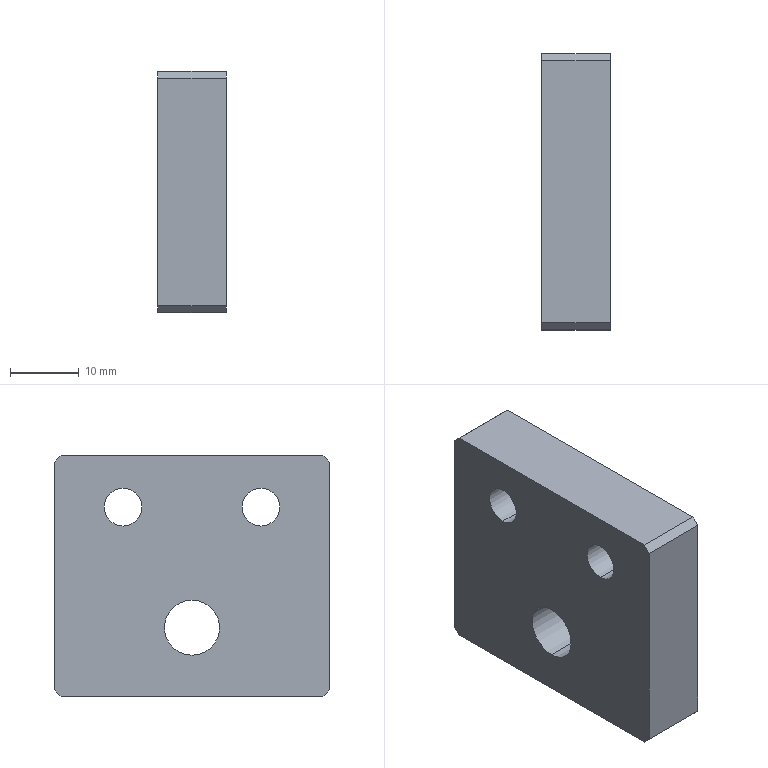Component | SolidWorks | XT-1-23-2-1 | 1 solid | 22 faces | box 10 x 40 x 35 mm | volume 12411 mm3 | plane 12 | cylinder 10 | commonest cylinder face diameters 10 x4 5.5 x4 8 x2
build123d program:
from build123d import *

# Parameters (mm, degrees)
SKETCH1_W                                       = 35
SKETCH1_H                                       = 40
BOSS_EXTRUDE1_DEPTH                             = 10
M5_HEX_SOCKET_HEAD_CAP_SCREW_CBORE1_D           = 5.5
M5_HEX_SOCKET_HEAD_CAP_SCREW_CBORE1_CBORE_D     = 10
M5_HEX_SOCKET_HEAD_CAP_SCREW_CBORE1_CBORE_DEPTH = 5.4
M8_TAPPED_HOLE1_D                               = 8
CHAMFER1_SIZE                                   = 1


with BuildPart() as part:
    # Sketch1 → Boss-Extrude1 (new body)
    with BuildSketch(Plane.XY):
        with Locations((17.5, -20)):
            Rectangle(SKETCH1_W, SKETCH1_H)
    extrude(amount=BOSS_EXTRUDE1_DEPTH)

    # M5 Hex Socket Head Cap Screw CBORE1 (through all)
    with Locations(Plane.XY.offset(10)):
        with Locations((7.5, -10), (7.5, -30)):
            CounterBoreHole(M5_HEX_SOCKET_HEAD_CAP_SCREW_CBORE1_D / 2, M5_HEX_SOCKET_HEAD_CAP_SCREW_CBORE1_CBORE_D / 2, M5_HEX_SOCKET_HEAD_CAP_SCREW_CBORE1_CBORE_DEPTH)

    # M8 Tapped Hole1 (through all)
    with Locations(Plane.XY.offset(10)):
        with Locations((25, -20)):
            Hole(M8_TAPPED_HOLE1_D / 2)

    # Chamfer1
    chamfer1_edges = [part.edges().sort_by_distance(p)[0] for p in [
        (0, 0, 5),
        (35, 0, 5),
        (35, -40, 5),
        (0, -40, 5),
    ]]
    chamfer(chamfer1_edges, length=CHAMFER1_SIZE)


solid = part.part

# Placed as in the assembly
solid = solid.moved(Location((587.283, -98.615, 20.5), (0, 90, 0)))
STEP:
#1=CARTESIAN_POINT('',(23.121,-4.67,-0.01969));
#2=VERTEX_POINT('',#1);
#3=CARTESIAN_POINT('',(23.121,-4.67,-0.3346));
#4=VERTEX_POINT('',#3);
#5=CARTESIAN_POINT('',(23.121,-4.67,-0.1772));
#6=DIRECTION('',(1.,-0.,0.));
#7=DIRECTION('',(0.,0.,-1.));
#8=AXIS2_PLACEMENT_3D('',#5,#6,#7);
#9=CIRCLE('',#8,0.1575);
#10=EDGE_CURVE('',#2,#4,#9,.T.);
#11=ORIENTED_EDGE('',*,*,#10,.F.);
#12=CARTESIAN_POINT('',(23.515,-4.67,-0.01969));
#13=VERTEX_POINT('',#12);
#14=CARTESIAN_POINT('',(23.515,-4.67,-0.01969));
#15=DIRECTION('',(1.,-0.,0.));
#16=VECTOR('',#15,39.37);
#17=LINE('',#14,#16);
#18=EDGE_CURVE('',#2,#13,#17,.T.);
#19=ORIENTED_EDGE('',*,*,#18,.T.);
#20=CARTESIAN_POINT('',(23.515,-4.67,-0.3346));
#21=VERTEX_POINT('',#20);
#22=CARTESIAN_POINT('',(23.515,-4.67,-0.1772));
#23=DIRECTION('',(1.,-0.,0.));
#24=DIRECTION('',(0.,0.,-1.));
#25=AXIS2_PLACEMENT_3D('',#22,#23,#24);
#26=CIRCLE('',#25,0.1575);
#27=EDGE_CURVE('',#13,#21,#26,.T.);
#28=ORIENTED_EDGE('',*,*,#27,.T.);
#29=CARTESIAN_POINT('',(23.515,-4.67,-0.3346));
#30=DIRECTION('',(1.,-0.,0.));
#31=VECTOR('',#30,39.37);
#32=LINE('',#29,#31);
#33=EDGE_CURVE('',#4,#21,#32,.T.);
#34=ORIENTED_EDGE('',*,*,#33,.F.);
#35=EDGE_LOOP('',(#11,#19,#28,#34));
#36=FACE_OUTER_BOUND('',#35,.T.);
#37=CARTESIAN_POINT('',(23.515,-4.67,-0.1772));
#38=DIRECTION('',(1.,-0.,0.));
#39=DIRECTION('',(0.,0.,-1.));
#40=AXIS2_PLACEMENT_3D('',#37,#38,#39);
#41=CYLINDRICAL_SURFACE('',#40,0.1575);
#42=ADVANCED_FACE('',(#36),#41,.F.);
#43=CARTESIAN_POINT('',(23.302,-4.276,0.7087));
#44=VERTEX_POINT('',#43);
#45=CARTESIAN_POINT('',(23.302,-4.276,0.315));
#46=VERTEX_POINT('',#45);
#47=CARTESIAN_POINT('',(23.302,-4.276,0.5118));
#48=DIRECTION('',(1.,-0.,0.));
#49=DIRECTION('',(0.,0.,-1.));
#50=AXIS2_PLACEMENT_3D('',#47,#48,#49);
#51=CIRCLE('',#50,0.1969);
#52=EDGE_CURVE('',#44,#46,#51,.T.);
#53=ORIENTED_EDGE('',*,*,#52,.F.);
#54=CARTESIAN_POINT('',(23.515,-4.276,0.7087));
#55=VERTEX_POINT('',#54);
#56=CARTESIAN_POINT('',(23.515,-4.276,0.7087));
#57=DIRECTION('',(1.,-0.,0.));
#58=VECTOR('',#57,39.37);
#59=LINE('',#56,#58);
#60=EDGE_CURVE('',#44,#55,#59,.T.);
#61=ORIENTED_EDGE('',*,*,#60,.T.);
#62=CARTESIAN_POINT('',(23.515,-4.276,0.315));
#63=VERTEX_POINT('',#62);
#64=CARTESIAN_POINT('',(23.515,-4.276,0.5118));
#65=DIRECTION('',(1.,-0.,0.));
#66=DIRECTION('',(0.,0.,-1.));
#67=AXIS2_PLACEMENT_3D('',#64,#65,#66);
#68=CIRCLE('',#67,0.1969);
#69=EDGE_CURVE('',#55,#63,#68,.T.);
#70=ORIENTED_EDGE('',*,*,#69,.T.);
#71=CARTESIAN_POINT('',(23.515,-4.276,0.315));
#72=DIRECTION('',(1.,-0.,0.));
#73=VECTOR('',#72,39.37);
#74=LINE('',#71,#73);
#75=EDGE_CURVE('',#46,#63,#74,.T.);
#76=ORIENTED_EDGE('',*,*,#75,.F.);
#77=EDGE_LOOP('',(#53,#61,#70,#76));
#78=FACE_OUTER_BOUND('',#77,.T.);
#79=CARTESIAN_POINT('',(23.515,-4.276,0.5118));
#80=DIRECTION('',(1.,-0.,0.));
#81=DIRECTION('',(0.,0.,-1.));
#82=AXIS2_PLACEMENT_3D('',#79,#80,#81);
#83=CYLINDRICAL_SURFACE('',#82,0.1969);
#84=ADVANCED_FACE('',(#78),#83,.F.);
#85=CARTESIAN_POINT('',(23.121,-4.276,0.6201));
#86=VERTEX_POINT('',#85);
#87=CARTESIAN_POINT('',(23.121,-4.276,0.4035));
#88=VERTEX_POINT('',#87);
#89=CARTESIAN_POINT('',(23.121,-4.276,0.5118));
#90=DIRECTION('',(1.,-0.,0.));
#91=DIRECTION('',(0.,0.,-1.));
#92=AXIS2_PLACEMENT_3D('',#89,#90,#91);
#93=CIRCLE('',#92,0.1083);
#94=EDGE_CURVE('',#86,#88,#93,.T.);
#95=ORIENTED_EDGE('',*,*,#94,.F.);
#96=CARTESIAN_POINT('',(23.302,-4.276,0.6201));
#97=VERTEX_POINT('',#96);
#98=CARTESIAN_POINT('',(23.515,-4.276,0.6201));
#99=DIRECTION('',(1.,-0.,0.));
#100=VECTOR('',#99,39.37);
#101=LINE('',#98,#100);
#102=EDGE_CURVE('',#86,#97,#101,.T.);
#103=ORIENTED_EDGE('',*,*,#102,.T.);
#104=CARTESIAN_POINT('',(23.302,-4.276,0.4035));
#105=VERTEX_POINT('',#104);
#106=CARTESIAN_POINT('',(23.302,-4.276,0.5118));
#107=DIRECTION('',(1.,-0.,0.));
#108=DIRECTION('',(0.,0.,-1.));
#109=AXIS2_PLACEMENT_3D('',#106,#107,#108);
#110=CIRCLE('',#109,0.1083);
#111=EDGE_CURVE('',#97,#105,#110,.T.);
#112=ORIENTED_EDGE('',*,*,#111,.T.);
#113=CARTESIAN_POINT('',(23.515,-4.276,0.4035));
#114=DIRECTION('',(1.,-0.,0.));
#115=VECTOR('',#114,39.37);
#116=LINE('',#113,#115);
#117=EDGE_CURVE('',#88,#105,#116,.T.);
#118=ORIENTED_EDGE('',*,*,#117,.F.);
#119=EDGE_LOOP('',(#95,#103,#112,#118));
#120=FACE_OUTER_BOUND('',#119,.T.);
#121=CARTESIAN_POINT('',(23.515,-4.276,0.5118));
#122=DIRECTION('',(1.,-0.,0.));
#123=DIRECTION('',(0.,0.,-1.));
#124=AXIS2_PLACEMENT_3D('',#121,#122,#123);
#125=CYLINDRICAL_SURFACE('',#124,0.1083);
#126=ADVANCED_FACE('',(#120),#125,.F.);
#127=CARTESIAN_POINT('',(23.302,-5.064,0.7087));
#128=VERTEX_POINT('',#127);
#129=CARTESIAN_POINT('',(23.302,-5.064,0.315));
#130=VERTEX_POINT('',#129);
#131=CARTESIAN_POINT('',(23.302,-5.064,0.5118));
#132=DIRECTION('',(1.,-0.,0.));
#133=DIRECTION('',(0.,0.,-1.));
#134=AXIS2_PLACEMENT_3D('',#131,#132,#133);
#135=CIRCLE('',#134,0.1969);
#136=EDGE_CURVE('',#128,#130,#135,.T.);
#137=ORIENTED_EDGE('',*,*,#136,.F.);
#138=CARTESIAN_POINT('',(23.515,-5.064,0.7087));
#139=VERTEX_POINT('',#138);
#140=CARTESIAN_POINT('',(23.515,-5.064,0.7087));
#141=DIRECTION('',(1.,-0.,0.));
#142=VECTOR('',#141,39.37);
#143=LINE('',#140,#142);
#144=EDGE_CURVE('',#128,#139,#143,.T.);
#145=ORIENTED_EDGE('',*,*,#144,.T.);
#146=CARTESIAN_POINT('',(23.515,-5.064,0.315));
#147=VERTEX_POINT('',#146);
#148=CARTESIAN_POINT('',(23.515,-5.064,0.5118));
#149=DIRECTION('',(1.,-0.,0.));
#150=DIRECTION('',(0.,0.,-1.));
#151=AXIS2_PLACEMENT_3D('',#148,#149,#150);
#152=CIRCLE('',#151,0.1969);
#153=EDGE_CURVE('',#139,#147,#152,.T.);
#154=ORIENTED_EDGE('',*,*,#153,.T.);
#155=CARTESIAN_POINT('',(23.515,-5.064,0.315));
#156=DIRECTION('',(1.,-0.,0.));
#157=VECTOR('',#156,39.37);
#158=LINE('',#155,#157);
#159=EDGE_CURVE('',#130,#147,#158,.T.);
#160=ORIENTED_EDGE('',*,*,#159,.F.);
#161=EDGE_LOOP('',(#137,#145,#154,#160));
#162=FACE_OUTER_BOUND('',#161,.T.);
#163=CARTESIAN_POINT('',(23.515,-5.064,0.5118));
#164=DIRECTION('',(1.,-0.,0.));
#165=DIRECTION('',(0.,0.,-1.));
#166=AXIS2_PLACEMENT_3D('',#163,#164,#165);
#167=CYLINDRICAL_SURFACE('',#166,0.1969);
#168=ADVANCED_FACE('',(#162),#167,.F.);
#169=CARTESIAN_POINT('',(23.121,-5.064,0.6201));
#170=VERTEX_POINT('',#169);
#171=CARTESIAN_POINT('',(23.121,-5.064,0.4035));
#172=VERTEX_POINT('',#171);
#173=CARTESIAN_POINT('',(23.121,-5.064,0.5118));
#174=DIRECTION('',(1.,-0.,0.));
#175=DIRECTION('',(0.,0.,-1.));
#176=AXIS2_PLACEMENT_3D('',#173,#174,#175);
#177=CIRCLE('',#176,0.1083);
#178=EDGE_CURVE('',#170,#172,#177,.T.);
#179=ORIENTED_EDGE('',*,*,#178,.F.);
#180=CARTESIAN_POINT('',(23.302,-5.064,0.6201));
#181=VERTEX_POINT('',#180);
#182=CARTESIAN_POINT('',(23.515,-5.064,0.6201));
#183=DIRECTION('',(1.,-0.,0.));
#184=VECTOR('',#183,39.37);
#185=LINE('',#182,#184);
#186=EDGE_CURVE('',#170,#181,#185,.T.);
#187=ORIENTED_EDGE('',*,*,#186,.T.);
#188=CARTESIAN_POINT('',(23.302,-5.064,0.4035));
#189=VERTEX_POINT('',#188);
#190=CARTESIAN_POINT('',(23.302,-5.064,0.5118));
#191=DIRECTION('',(1.,-0.,0.));
#192=DIRECTION('',(0.,0.,-1.));
#193=AXIS2_PLACEMENT_3D('',#190,#191,#192);
#194=CIRCLE('',#193,0.1083);
#195=EDGE_CURVE('',#181,#189,#194,.T.);
#196=ORIENTED_EDGE('',*,*,#195,.T.);
#197=CARTESIAN_POINT('',(23.515,-5.064,0.4035));
#198=DIRECTION('',(1.,-0.,0.));
#199=VECTOR('',#198,39.37);
#200=LINE('',#197,#199);
#201=EDGE_CURVE('',#172,#189,#200,.T.);
#202=ORIENTED_EDGE('',*,*,#201,.F.);
#203=EDGE_LOOP('',(#179,#187,#196,#202));
#204=FACE_OUTER_BOUND('',#203,.T.);
#205=CARTESIAN_POINT('',(23.515,-5.064,0.5118));
#206=DIRECTION('',(1.,-0.,0.));
#207=DIRECTION('',(0.,0.,-1.));
#208=AXIS2_PLACEMENT_3D('',#205,#206,#207);
#209=CYLINDRICAL_SURFACE('',#208,0.1083);
#210=ADVANCED_FACE('',(#204),#209,.F.);
#211=CARTESIAN_POINT('',(23.121,-3.922,0.8071));
#212=VERTEX_POINT('',#211);
#213=CARTESIAN_POINT('',(23.121,-5.418,0.8071));
#214=VERTEX_POINT('',#213);
#215=CARTESIAN_POINT('',(23.121,-3.882,0.8071));
#216=DIRECTION('',(-0.,-1.,-0.));
#217=VECTOR('',#216,39.37);
#218=LINE('',#215,#217);
#219=EDGE_CURVE('',#212,#214,#218,.T.);
#220=ORIENTED_EDGE('',*,*,#219,.T.);
#221=CARTESIAN_POINT('',(23.515,-5.418,0.8071));
#222=VERTEX_POINT('',#221);
#223=CARTESIAN_POINT('',(23.515,-5.418,0.8071));
#224=DIRECTION('',(1.,-0.,0.));
#225=VECTOR('',#224,39.37);
#226=LINE('',#223,#225);
#227=EDGE_CURVE('',#214,#222,#226,.T.);
#228=ORIENTED_EDGE('',*,*,#227,.T.);
#229=CARTESIAN_POINT('',(23.515,-3.922,0.8071));
#230=VERTEX_POINT('',#229);
#231=CARTESIAN_POINT('',(23.515,-3.882,0.8071));
#232=DIRECTION('',(-0.,-1.,-0.));
#233=VECTOR('',#232,39.37);
#234=LINE('',#231,#233);
#235=EDGE_CURVE('',#230,#222,#234,.T.);
#236=ORIENTED_EDGE('',*,*,#235,.F.);
#237=CARTESIAN_POINT('',(23.515,-3.922,0.8071));
#238=DIRECTION('',(-1.,0.,0.));
#239=VECTOR('',#238,39.37);
#240=LINE('',#237,#239);
#241=EDGE_CURVE('',#230,#212,#240,.T.);
#242=ORIENTED_EDGE('',*,*,#241,.T.);
#243=EDGE_LOOP('',(#220,#228,#236,#242));
#244=FACE_OUTER_BOUND('',#243,.T.);
#245=CARTESIAN_POINT('',(23.515,-3.882,0.8071));
#246=DIRECTION('',(0.,0.,-1.));
#247=DIRECTION('',(0.,1.,0.));
#248=AXIS2_PLACEMENT_3D('',#245,#246,#247);
#249=PLANE('',#248);
#250=ADVANCED_FACE('',(#244),#249,.F.);
#251=CARTESIAN_POINT('',(23.515,-5.457,0.7677));
#252=VERTEX_POINT('',#251);
#253=CARTESIAN_POINT('',(23.515,-5.457,-0.5315));
#254=VERTEX_POINT('',#253);
#255=CARTESIAN_POINT('',(23.515,-5.457,0.8071));
#256=DIRECTION('',(0.,0.,-1.));
#257=VECTOR('',#256,39.37);
#258=LINE('',#255,#257);
#259=EDGE_CURVE('',#252,#254,#258,.T.);
#260=ORIENTED_EDGE('',*,*,#259,.F.);
#261=CARTESIAN_POINT('',(23.121,-5.457,0.7677));
#262=VERTEX_POINT('',#261);
#263=CARTESIAN_POINT('',(23.515,-5.457,0.7677));
#264=DIRECTION('',(-1.,0.,0.));
#265=VECTOR('',#264,39.37);
#266=LINE('',#263,#265);
#267=EDGE_CURVE('',#252,#262,#266,.T.);
#268=ORIENTED_EDGE('',*,*,#267,.T.);
#269=CARTESIAN_POINT('',(23.121,-5.457,-0.5315));
#270=VERTEX_POINT('',#269);
#271=CARTESIAN_POINT('',(23.121,-5.457,0.8071));
#272=DIRECTION('',(0.,0.,-1.));
#273=VECTOR('',#272,39.37);
#274=LINE('',#271,#273);
#275=EDGE_CURVE('',#262,#270,#274,.T.);
#276=ORIENTED_EDGE('',*,*,#275,.T.);
#277=CARTESIAN_POINT('',(23.515,-5.457,-0.5315));
#278=DIRECTION('',(1.,-0.,0.));
#279=VECTOR('',#278,39.37);
#280=LINE('',#277,#279);
#281=EDGE_CURVE('',#270,#254,#280,.T.);
#282=ORIENTED_EDGE('',*,*,#281,.T.);
#283=EDGE_LOOP('',(#260,#268,#276,#282));
#284=FACE_OUTER_BOUND('',#283,.T.);
#285=CARTESIAN_POINT('',(23.515,-5.457,0.8071));
#286=DIRECTION('',(0.,1.,0.));
#287=DIRECTION('',(1.,-0.,0.));
#288=AXIS2_PLACEMENT_3D('',#285,#286,#287);
#289=PLANE('',#288);
#290=ADVANCED_FACE('',(#284),#289,.F.);
#291=CARTESIAN_POINT('',(23.515,-5.418,-0.5709));
#292=VERTEX_POINT('',#291);
#293=CARTESIAN_POINT('',(23.515,-3.922,-0.5709));
#294=VERTEX_POINT('',#293);
#295=CARTESIAN_POINT('',(23.515,-3.882,-0.5709));
#296=DIRECTION('',(0.,1.,0.));
#297=VECTOR('',#296,39.37);
#298=LINE('',#295,#297);
#299=EDGE_CURVE('',#292,#294,#298,.T.);
#300=ORIENTED_EDGE('',*,*,#299,.F.);
#301=CARTESIAN_POINT('',(23.121,-5.418,-0.5709));
#302=VERTEX_POINT('',#301);
#303=CARTESIAN_POINT('',(23.515,-5.418,-0.5709));
#304=DIRECTION('',(-1.,0.,0.));
#305=VECTOR('',#304,39.37);
#306=LINE('',#303,#305);
#307=EDGE_CURVE('',#292,#302,#306,.T.);
#308=ORIENTED_EDGE('',*,*,#307,.T.);
#309=CARTESIAN_POINT('',(23.121,-3.922,-0.5709));
#310=VERTEX_POINT('',#309);
#311=CARTESIAN_POINT('',(23.121,-3.882,-0.5709));
#312=DIRECTION('',(0.,1.,0.));
#313=VECTOR('',#312,39.37);
#314=LINE('',#311,#313);
#315=EDGE_CURVE('',#302,#310,#314,.T.);
#316=ORIENTED_EDGE('',*,*,#315,.T.);
#317=CARTESIAN_POINT('',(23.515,-3.922,-0.5709));
#318=DIRECTION('',(1.,-0.,0.));
#319=VECTOR('',#318,39.37);
#320=LINE('',#317,#319);
#321=EDGE_CURVE('',#310,#294,#320,.T.);
#322=ORIENTED_EDGE('',*,*,#321,.T.);
#323=EDGE_LOOP('',(#300,#308,#316,#322));
#324=FACE_OUTER_BOUND('',#323,.T.);
#325=CARTESIAN_POINT('',(23.515,-3.882,-0.5709));
#326=DIRECTION('',(-0.,-0.,1.));
#327=DIRECTION('',(-0.,-1.,-0.));
#328=AXIS2_PLACEMENT_3D('',#325,#326,#327);
#329=PLANE('',#328);
#330=ADVANCED_FACE('',(#324),#329,.F.);
#331=CARTESIAN_POINT('',(23.515,-3.882,-0.5315));
#332=VERTEX_POINT('',#331);
#333=CARTESIAN_POINT('',(23.515,-3.882,0.7677));
#334=VERTEX_POINT('',#333);
#335=CARTESIAN_POINT('',(23.515,-3.882,0.8071));
#336=DIRECTION('',(-0.,-0.,1.));
#337=VECTOR('',#336,39.37);
#338=LINE('',#335,#337);
#339=EDGE_CURVE('',#332,#334,#338,.T.);
#340=ORIENTED_EDGE('',*,*,#339,.F.);
#341=CARTESIAN_POINT('',(23.121,-3.882,-0.5315));
#342=VERTEX_POINT('',#341);
#343=CARTESIAN_POINT('',(23.515,-3.882,-0.5315));
#344=DIRECTION('',(-1.,0.,0.));
#345=VECTOR('',#344,39.37);
#346=LINE('',#343,#345);
#347=EDGE_CURVE('',#332,#342,#346,.T.);
#348=ORIENTED_EDGE('',*,*,#347,.T.);
#349=CARTESIAN_POINT('',(23.121,-3.882,0.7677));
#350=VERTEX_POINT('',#349);
#351=CARTESIAN_POINT('',(23.121,-3.882,0.8071));
#352=DIRECTION('',(-0.,-0.,1.));
#353=VECTOR('',#352,39.37);
#354=LINE('',#351,#353);
#355=EDGE_CURVE('',#342,#350,#354,.T.);
#356=ORIENTED_EDGE('',*,*,#355,.T.);
#357=CARTESIAN_POINT('',(23.515,-3.882,0.7677));
#358=DIRECTION('',(1.,-0.,0.));
#359=VECTOR('',#358,39.37);
#360=LINE('',#357,#359);
#361=EDGE_CURVE('',#350,#334,#360,.T.);
#362=ORIENTED_EDGE('',*,*,#361,.T.);
#363=EDGE_LOOP('',(#340,#348,#356,#362));
#364=FACE_OUTER_BOUND('',#363,.T.);
#365=CARTESIAN_POINT('',(23.515,-3.882,0.8071));
#366=DIRECTION('',(-0.,-1.,-0.));
#367=DIRECTION('',(-1.,0.,0.));
#368=AXIS2_PLACEMENT_3D('',#365,#366,#367);
#369=PLANE('',#368);
#370=ADVANCED_FACE('',(#364),#369,.F.);
#371=CARTESIAN_POINT('',(23.515,-4.67,-0.1772));
#372=DIRECTION('',(1.,-0.,0.));
#373=DIRECTION('',(0.,0.,-1.));
#374=AXIS2_PLACEMENT_3D('',#371,#372,#373);
#375=CIRCLE('',#374,0.1575);
#376=EDGE_CURVE('',#21,#13,#375,.T.);
#377=ORIENTED_EDGE('',*,*,#376,.F.);
#378=ORIENTED_EDGE('',*,*,#27,.F.);
#379=EDGE_LOOP('',(#377,#378));
#380=FACE_BOUND('',#379,.T.);
#381=CARTESIAN_POINT('',(23.515,-4.276,0.5118));
#382=DIRECTION('',(1.,-0.,0.));
#383=DIRECTION('',(0.,0.,-1.));
#384=AXIS2_PLACEMENT_3D('',#381,#382,#383);
#385=CIRCLE('',#384,0.1969);
#386=EDGE_CURVE('',#63,#55,#385,.T.);
#387=ORIENTED_EDGE('',*,*,#386,.F.);
#388=ORIENTED_EDGE('',*,*,#69,.F.);
#389=EDGE_LOOP('',(#387,#388));
#390=FACE_BOUND('',#389,.T.);
#391=CARTESIAN_POINT('',(23.515,-5.064,0.5118));
#392=DIRECTION('',(1.,-0.,0.));
#393=DIRECTION('',(0.,0.,-1.));
#394=AXIS2_PLACEMENT_3D('',#391,#392,#393);
#395=CIRCLE('',#394,0.1969);
#396=EDGE_CURVE('',#147,#139,#395,.T.);
#397=ORIENTED_EDGE('',*,*,#396,.F.);
#398=ORIENTED_EDGE('',*,*,#153,.F.);
#399=EDGE_LOOP('',(#397,#398));
#400=FACE_BOUND('',#399,.T.);
#401=ORIENTED_EDGE('',*,*,#235,.T.);
#402=CARTESIAN_POINT('',(23.515,-4.65,1.575));
#403=DIRECTION('',(-0.,-0.7071,-0.7071));
#404=VECTOR('',#403,39.37);
#405=LINE('',#402,#404);
#406=EDGE_CURVE('',#222,#252,#405,.T.);
#407=ORIENTED_EDGE('',*,*,#406,.T.);
#408=ORIENTED_EDGE('',*,*,#259,.T.);
#409=CARTESIAN_POINT('',(23.515,-5.339,-0.6496));
#410=DIRECTION('',(0.,0.7071,-0.7071));
#411=VECTOR('',#410,39.37);
#412=LINE('',#409,#411);
#413=EDGE_CURVE('',#254,#292,#412,.T.);
#414=ORIENTED_EDGE('',*,*,#413,.T.);
#415=ORIENTED_EDGE('',*,*,#299,.T.);
#416=CARTESIAN_POINT('',(23.515,-3.213,0.1378));
#417=DIRECTION('',(0.,0.7071,0.7071));
#418=VECTOR('',#417,39.37);
#419=LINE('',#416,#418);
#420=EDGE_CURVE('',#294,#332,#419,.T.);
#421=ORIENTED_EDGE('',*,*,#420,.T.);
#422=ORIENTED_EDGE('',*,*,#339,.T.);
#423=CARTESIAN_POINT('',(23.515,-3.902,0.7874));
#424=DIRECTION('',(-0.,-0.7071,0.7071));
#425=VECTOR('',#424,39.37);
#426=LINE('',#423,#425);
#427=EDGE_CURVE('',#334,#230,#426,.T.);
#428=ORIENTED_EDGE('',*,*,#427,.T.);
#429=EDGE_LOOP('',(#401,#407,#408,#414,#415,#421,#422,#428));
#430=FACE_OUTER_BOUND('',#429,.T.);
#431=CARTESIAN_POINT('',(23.515,-3.882,0.8071));
#432=DIRECTION('',(1.,-0.,0.));
#433=DIRECTION('',(0.,0.,-1.));
#434=AXIS2_PLACEMENT_3D('',#431,#432,#433);
#435=PLANE('',#434);
#436=ADVANCED_FACE('',(#380,#390,#400,#430),#435,.T.);
#437=CARTESIAN_POINT('',(23.121,-4.67,-0.1772));
#438=DIRECTION('',(1.,-0.,0.));
#439=DIRECTION('',(0.,0.,-1.));
#440=AXIS2_PLACEMENT_3D('',#437,#438,#439);
#441=CIRCLE('',#440,0.1575);
#442=EDGE_CURVE('',#4,#2,#441,.T.);
#443=ORIENTED_EDGE('',*,*,#442,.T.);
#444=ORIENTED_EDGE('',*,*,#10,.T.);
#445=EDGE_LOOP('',(#443,#444));
#446=FACE_BOUND('',#445,.T.);
#447=CARTESIAN_POINT('',(23.121,-4.276,0.5118));
#448=DIRECTION('',(1.,-0.,0.));
#449=DIRECTION('',(0.,0.,-1.));
#450=AXIS2_PLACEMENT_3D('',#447,#448,#449);
#451=CIRCLE('',#450,0.1083);
#452=EDGE_CURVE('',#88,#86,#451,.T.);
#453=ORIENTED_EDGE('',*,*,#452,.T.);
#454=ORIENTED_EDGE('',*,*,#94,.T.);
#455=EDGE_LOOP('',(#453,#454));
#456=FACE_BOUND('',#455,.T.);
#457=CARTESIAN_POINT('',(23.121,-5.064,0.5118));
#458=DIRECTION('',(1.,-0.,0.));
#459=DIRECTION('',(0.,0.,-1.));
#460=AXIS2_PLACEMENT_3D('',#457,#458,#459);
#461=CIRCLE('',#460,0.1083);
#462=EDGE_CURVE('',#172,#170,#461,.T.);
#463=ORIENTED_EDGE('',*,*,#462,.T.);
#464=ORIENTED_EDGE('',*,*,#178,.T.);
#465=EDGE_LOOP('',(#463,#464));
#466=FACE_BOUND('',#465,.T.);
#467=ORIENTED_EDGE('',*,*,#275,.F.);
#468=CARTESIAN_POINT('',(23.121,-5.457,0.7677));
#469=DIRECTION('',(0.,0.7071,0.7071));
#470=VECTOR('',#469,39.37);
#471=LINE('',#468,#470);
#472=EDGE_CURVE('',#262,#214,#471,.T.);
#473=ORIENTED_EDGE('',*,*,#472,.T.);
#474=ORIENTED_EDGE('',*,*,#219,.F.);
#475=CARTESIAN_POINT('',(23.121,-3.922,0.8071));
#476=DIRECTION('',(0.,0.7071,-0.7071));
#477=VECTOR('',#476,39.37);
#478=LINE('',#475,#477);
#479=EDGE_CURVE('',#212,#350,#478,.T.);
#480=ORIENTED_EDGE('',*,*,#479,.T.);
#481=ORIENTED_EDGE('',*,*,#355,.F.);
#482=CARTESIAN_POINT('',(23.121,-3.882,-0.5315));
#483=DIRECTION('',(-0.,-0.7071,-0.7071));
#484=VECTOR('',#483,39.37);
#485=LINE('',#482,#484);
#486=EDGE_CURVE('',#342,#310,#485,.T.);
#487=ORIENTED_EDGE('',*,*,#486,.T.);
#488=ORIENTED_EDGE('',*,*,#315,.F.);
#489=CARTESIAN_POINT('',(23.121,-5.418,-0.5709));
#490=DIRECTION('',(-0.,-0.7071,0.7071));
#491=VECTOR('',#490,39.37);
#492=LINE('',#489,#491);
#493=EDGE_CURVE('',#302,#270,#492,.T.);
#494=ORIENTED_EDGE('',*,*,#493,.T.);
#495=EDGE_LOOP('',(#467,#473,#474,#480,#481,#487,#488,#494));
#496=FACE_OUTER_BOUND('',#495,.T.);
#497=CARTESIAN_POINT('',(23.121,-3.882,0.8071));
#498=DIRECTION('',(1.,-0.,0.));
#499=DIRECTION('',(0.,0.,-1.));
#500=AXIS2_PLACEMENT_3D('',#497,#498,#499);
#501=PLANE('',#500);
#502=ADVANCED_FACE('',(#446,#456,#466,#496),#501,.F.);
#503=ORIENTED_EDGE('',*,*,#186,.F.);
#504=ORIENTED_EDGE('',*,*,#462,.F.);
#505=ORIENTED_EDGE('',*,*,#201,.T.);
#506=CARTESIAN_POINT('',(23.302,-5.064,0.5118));
#507=DIRECTION('',(1.,-0.,0.));
#508=DIRECTION('',(0.,0.,-1.));
#509=AXIS2_PLACEMENT_3D('',#506,#507,#508);
#510=CIRCLE('',#509,0.1083);
#511=EDGE_CURVE('',#189,#181,#510,.T.);
#512=ORIENTED_EDGE('',*,*,#511,.T.);
#513=EDGE_LOOP('',(#503,#504,#505,#512));
#514=FACE_OUTER_BOUND('',#513,.T.);
#515=CARTESIAN_POINT('',(23.515,-5.064,0.5118));
#516=DIRECTION('',(1.,-0.,0.));
#517=DIRECTION('',(0.,0.,-1.));
#518=AXIS2_PLACEMENT_3D('',#515,#516,#517);
#519=CYLINDRICAL_SURFACE('',#518,0.1083);
#520=ADVANCED_FACE('',(#514),#519,.F.);
#521=ORIENTED_EDGE('',*,*,#511,.F.);
#522=ORIENTED_EDGE('',*,*,#195,.F.);
#523=EDGE_LOOP('',(#521,#522));
#524=FACE_BOUND('',#523,.T.);
#525=CARTESIAN_POINT('',(23.302,-5.064,0.5118));
#526=DIRECTION('',(1.,-0.,0.));
#527=DIRECTION('',(0.,0.,-1.));
#528=AXIS2_PLACEMENT_3D('',#525,#526,#527);
#529=CIRCLE('',#528,0.1969);
#530=EDGE_CURVE('',#130,#128,#529,.T.);
#531=ORIENTED_EDGE('',*,*,#530,.T.);
#532=ORIENTED_EDGE('',*,*,#136,.T.);
#533=EDGE_LOOP('',(#531,#532));
#534=FACE_OUTER_BOUND('',#533,.T.);
#535=CARTESIAN_POINT('',(23.302,-5.064,0.4035));
#536=DIRECTION('',(-1.,0.,-0.));
#537=DIRECTION('',(-0.,-0.,1.));
#538=AXIS2_PLACEMENT_3D('',#535,#536,#537);
#539=PLANE('',#538);
#540=ADVANCED_FACE('',(#524,#534),#539,.F.);
#541=ORIENTED_EDGE('',*,*,#144,.F.);
#542=ORIENTED_EDGE('',*,*,#530,.F.);
#543=ORIENTED_EDGE('',*,*,#159,.T.);
#544=ORIENTED_EDGE('',*,*,#396,.T.);
#545=EDGE_LOOP('',(#541,#542,#543,#544));
#546=FACE_OUTER_BOUND('',#545,.T.);
#547=CARTESIAN_POINT('',(23.515,-5.064,0.5118));
#548=DIRECTION('',(1.,-0.,0.));
#549=DIRECTION('',(0.,0.,-1.));
#550=AXIS2_PLACEMENT_3D('',#547,#548,#549);
#551=CYLINDRICAL_SURFACE('',#550,0.1969);
#552=ADVANCED_FACE('',(#546),#551,.F.);
#553=ORIENTED_EDGE('',*,*,#102,.F.);
#554=ORIENTED_EDGE('',*,*,#452,.F.);
#555=ORIENTED_EDGE('',*,*,#117,.T.);
#556=CARTESIAN_POINT('',(23.302,-4.276,0.5118));
#557=DIRECTION('',(1.,-0.,0.));
#558=DIRECTION('',(0.,0.,-1.));
#559=AXIS2_PLACEMENT_3D('',#556,#557,#558);
#560=CIRCLE('',#559,0.1083);
#561=EDGE_CURVE('',#105,#97,#560,.T.);
#562=ORIENTED_EDGE('',*,*,#561,.T.);
#563=EDGE_LOOP('',(#553,#554,#555,#562));
#564=FACE_OUTER_BOUND('',#563,.T.);
#565=CARTESIAN_POINT('',(23.515,-4.276,0.5118));
#566=DIRECTION('',(1.,-0.,0.));
#567=DIRECTION('',(0.,0.,-1.));
#568=AXIS2_PLACEMENT_3D('',#565,#566,#567);
#569=CYLINDRICAL_SURFACE('',#568,0.1083);
#570=ADVANCED_FACE('',(#564),#569,.F.);
#571=ORIENTED_EDGE('',*,*,#561,.F.);
#572=ORIENTED_EDGE('',*,*,#111,.F.);
#573=EDGE_LOOP('',(#571,#572));
#574=FACE_BOUND('',#573,.T.);
#575=CARTESIAN_POINT('',(23.302,-4.276,0.5118));
#576=DIRECTION('',(1.,-0.,0.));
#577=DIRECTION('',(0.,0.,-1.));
#578=AXIS2_PLACEMENT_3D('',#575,#576,#577);
#579=CIRCLE('',#578,0.1969);
#580=EDGE_CURVE('',#46,#44,#579,.T.);
#581=ORIENTED_EDGE('',*,*,#580,.T.);
#582=ORIENTED_EDGE('',*,*,#52,.T.);
#583=EDGE_LOOP('',(#581,#582));
#584=FACE_OUTER_BOUND('',#583,.T.);
#585=CARTESIAN_POINT('',(23.302,-4.276,0.4035));
#586=DIRECTION('',(-1.,0.,-0.));
#587=DIRECTION('',(-0.,-0.,1.));
#588=AXIS2_PLACEMENT_3D('',#585,#586,#587);
#589=PLANE('',#588);
#590=ADVANCED_FACE('',(#574,#584),#589,.F.);
#591=ORIENTED_EDGE('',*,*,#60,.F.);
#592=ORIENTED_EDGE('',*,*,#580,.F.);
#593=ORIENTED_EDGE('',*,*,#75,.T.);
#594=ORIENTED_EDGE('',*,*,#386,.T.);
#595=EDGE_LOOP('',(#591,#592,#593,#594));
#596=FACE_OUTER_BOUND('',#595,.T.);
#597=CARTESIAN_POINT('',(23.515,-4.276,0.5118));
#598=DIRECTION('',(1.,-0.,0.));
#599=DIRECTION('',(0.,0.,-1.));
#600=AXIS2_PLACEMENT_3D('',#597,#598,#599);
#601=CYLINDRICAL_SURFACE('',#600,0.1969);
#602=ADVANCED_FACE('',(#596),#601,.F.);
#603=ORIENTED_EDGE('',*,*,#18,.F.);
#604=ORIENTED_EDGE('',*,*,#442,.F.);
#605=ORIENTED_EDGE('',*,*,#33,.T.);
#606=ORIENTED_EDGE('',*,*,#376,.T.);
#607=EDGE_LOOP('',(#603,#604,#605,#606));
#608=FACE_OUTER_BOUND('',#607,.T.);
#609=CARTESIAN_POINT('',(23.515,-4.67,-0.1772));
#610=DIRECTION('',(1.,-0.,0.));
#611=DIRECTION('',(0.,0.,-1.));
#612=AXIS2_PLACEMENT_3D('',#609,#610,#611);
#613=CYLINDRICAL_SURFACE('',#612,0.1575);
#614=ADVANCED_FACE('',(#608),#613,.F.);
#615=ORIENTED_EDGE('',*,*,#406,.F.);
#616=ORIENTED_EDGE('',*,*,#227,.F.);
#617=ORIENTED_EDGE('',*,*,#472,.F.);
#618=ORIENTED_EDGE('',*,*,#267,.F.);
#619=EDGE_LOOP('',(#615,#616,#617,#618));
#620=FACE_OUTER_BOUND('',#619,.T.);
#621=CARTESIAN_POINT('',(23.515,-5.457,0.7677));
#622=DIRECTION('',(0.,0.7071,-0.7071));
#623=DIRECTION('',(-1.,0.,0.));
#624=AXIS2_PLACEMENT_3D('',#621,#622,#623);
#625=PLANE('',#624);
#626=ADVANCED_FACE('',(#620),#625,.F.);
#627=ORIENTED_EDGE('',*,*,#413,.F.);
#628=ORIENTED_EDGE('',*,*,#281,.F.);
#629=ORIENTED_EDGE('',*,*,#493,.F.);
#630=ORIENTED_EDGE('',*,*,#307,.F.);
#631=EDGE_LOOP('',(#627,#628,#629,#630));
#632=FACE_OUTER_BOUND('',#631,.T.);
#633=CARTESIAN_POINT('',(23.515,-5.418,-0.5709));
#634=DIRECTION('',(0.,0.7071,0.7071));
#635=DIRECTION('',(-1.,0.,0.));
#636=AXIS2_PLACEMENT_3D('',#633,#634,#635);
#637=PLANE('',#636);
#638=ADVANCED_FACE('',(#632),#637,.F.);
#639=ORIENTED_EDGE('',*,*,#420,.F.);
#640=ORIENTED_EDGE('',*,*,#321,.F.);
#641=ORIENTED_EDGE('',*,*,#486,.F.);
#642=ORIENTED_EDGE('',*,*,#347,.F.);
#643=EDGE_LOOP('',(#639,#640,#641,#642));
#644=FACE_OUTER_BOUND('',#643,.T.);
#645=CARTESIAN_POINT('',(23.515,-3.882,-0.5315));
#646=DIRECTION('',(-0.,-0.7071,0.7071));
#647=DIRECTION('',(-1.,0.,0.));
#648=AXIS2_PLACEMENT_3D('',#645,#646,#647);
#649=PLANE('',#648);
#650=ADVANCED_FACE('',(#644),#649,.F.);
#651=ORIENTED_EDGE('',*,*,#427,.F.);
#652=ORIENTED_EDGE('',*,*,#361,.F.);
#653=ORIENTED_EDGE('',*,*,#479,.F.);
#654=ORIENTED_EDGE('',*,*,#241,.F.);
#655=EDGE_LOOP('',(#651,#652,#653,#654));
#656=FACE_OUTER_BOUND('',#655,.T.);
#657=CARTESIAN_POINT('',(23.515,-3.922,0.8071));
#658=DIRECTION('',(-0.,-0.7071,-0.7071));
#659=DIRECTION('',(-1.,0.,0.));
#660=AXIS2_PLACEMENT_3D('',#657,#658,#659);
#661=PLANE('',#660);
#662=ADVANCED_FACE('',(#656),#661,.F.);
#663=CLOSED_SHELL('',(#42,#84,#126,#168,#210,#250,#290,#330,#370,#436,#502,#520,#540,#552,#570,#590,#602,#614,#626,#638,#650,#662));
#664=MANIFOLD_SOLID_BREP('',#663);
#665=CARTESIAN_POINT('',(0.,0.,0.));
#666=DIRECTION('',(0.,0.,1.));
#667=DIRECTION('',(1.,0.,0.));
#668=AXIS2_PLACEMENT_3D('',#665,#666,#667);
#669=(LENGTH_UNIT()NAMED_UNIT(*)SI_UNIT($,.METRE.));
#670=LENGTH_MEASURE_WITH_UNIT(LENGTH_MEASURE(0.0254),#669);
#671=DIMENSIONAL_EXPONENTS(1.,0.,0.,0.,0.,0.,0.);
#672=(CONVERSION_BASED_UNIT('',#670)LENGTH_UNIT()NAMED_UNIT(#671));
#673=UNCERTAINTY_MEASURE_WITH_UNIT(LENGTH_MEASURE(0.00001),#672,'','');
#674=(NAMED_UNIT(*)PLANE_ANGLE_UNIT()SI_UNIT($,.RADIAN.));
#675=(NAMED_UNIT(*)SI_UNIT($,.STERADIAN.)SOLID_ANGLE_UNIT());
#676=(GEOMETRIC_REPRESENTATION_CONTEXT(3)GLOBAL_UNCERTAINTY_ASSIGNED_CONTEXT((#673))GLOBAL_UNIT_ASSIGNED_CONTEXT((#672,#674,#675))REPRESENTATION_CONTEXT('',''));
#677=ADVANCED_BREP_SHAPE_REPRESENTATION('',(#664,#668),#676);
#678=COLOUR_RGB('',0.7922,0.8196,0.9333);
#679=FILL_AREA_STYLE_COLOUR('',#678);
#680=FILL_AREA_STYLE('',(#679));
#681=SURFACE_STYLE_FILL_AREA(#680);
#682=SURFACE_SIDE_STYLE('',(#681));
#683=SURFACE_STYLE_USAGE(.BOTH.,#682);
#684=PRESENTATION_STYLE_ASSIGNMENT((#683));
#685=STYLED_ITEM('',(#684),#664);
#686=PRESENTATION_LAYER_ASSIGNMENT('','',(#685));
#687=(LENGTH_UNIT()NAMED_UNIT(*)SI_UNIT($,.METRE.));
#688=LENGTH_MEASURE_WITH_UNIT(LENGTH_MEASURE(0.0254),#687);
#689=DIMENSIONAL_EXPONENTS(1.,0.,0.,0.,0.,0.,0.);
#690=(CONVERSION_BASED_UNIT('',#688)LENGTH_UNIT()NAMED_UNIT(#689));
#691=UNCERTAINTY_MEASURE_WITH_UNIT(LENGTH_MEASURE(0.00001),#690,'','');
#692=(NAMED_UNIT(*)PLANE_ANGLE_UNIT()SI_UNIT($,.RADIAN.));
#693=(NAMED_UNIT(*)SI_UNIT($,.STERADIAN.)SOLID_ANGLE_UNIT());
#694=(GEOMETRIC_REPRESENTATION_CONTEXT(3)GLOBAL_UNCERTAINTY_ASSIGNED_CONTEXT((#691))GLOBAL_UNIT_ASSIGNED_CONTEXT((#690,#692,#693))REPRESENTATION_CONTEXT('',''));
#695=MECHANICAL_DESIGN_GEOMETRIC_PRESENTATION_REPRESENTATION('',(#685),#694);